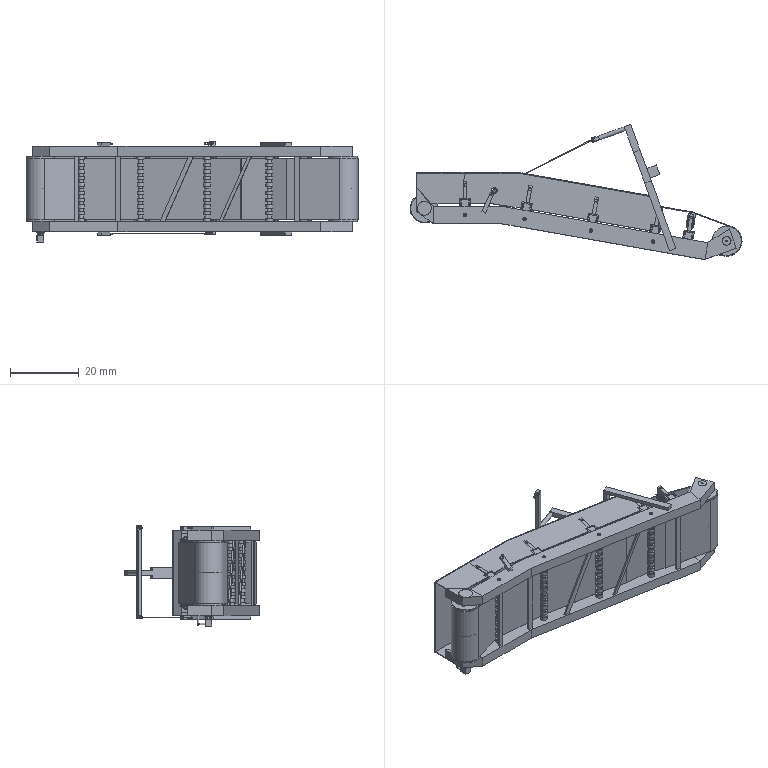Assembly | NX | mm | 27 component files | 141 solids | 1975 faces | box 96.68 x 39.38 x 29.23 mm | volume 7757 mm3 | plane 937 | cylinder 487 | cone 445 | sphere 86 | spline 14 | torus 6 | commonest cylinder face diameters 0.08 x104 0.1 x58 1.2 x41 2 x40 2.065 x35 1.51 x35 0.086 x27 0.8 x26
Bill of materials:
unnamed part 1 | 1 |  | Stepped solid cylinder: a larger central cylindrical body with a smaller coaxial cylindrical stub at each end.
unnamed part 2 | 5 |  | Rectangular open frame made of bar stock, with a long double-rib channel-like spine on one side, a fork-shaped connector at the ends, and a segmented, ribbed cylindrical member that bends in a shallow V/zigzag between the frame ends.
unnamed part 3 | 1 |  | Open framework of rectangular bars: a straight bar with small holes near both ends, joined by a stepped round/rectangular rod-and-block linkage to a C-shaped (three-sided) bar frame.
unnamed part 4 | 4 |  | Linked assembly-like shape: a U-bent round rod (hairpin loop) passes through a rectangular frame made of two flat bar plates joined by two round cross rods; a small pin is visible at the loop.
unnamed part 5 | 1 |  | Stepped cylinder: a large central cylindrical body with a smaller coaxial cylindrical stub at each end and a small axial hole through the center.
unnamed part 6 | 8 |  | Plain cylindrical sleeve/bushing-like tube with a concentric through-bore and flat ends.
unnamed part 7 | 4 |  | Slender stepped shaft with a regular series of evenly spaced larger-diameter collars/discs along its length, and stepped reduced-diameter ends.
unnamed part 8 | 1 |  | Long welded-frame-like structure of two parallel side plates with an angled (kinked) profile, joined by thin cross rods/bars and a solid web; it has round pivot holes at both ends, small holes, and stepped slot/notch features along the plates.
unnamed part 9 | 1 |  | Rectangular block body with stepped, smaller rectangular tiers on top, capped by a thin square flange plate with four corner holes and a larger central hole; two round rods leave the side, bend 90 degrees, and run upward parallel to each other.
unnamed part 10 | 1 |  | Thin-walled closed loop band: an elongated, slightly curved, rounded-end ring/strap profile extruded to a constant height, open on both faces.
Mates:
1. touch align | assembly face | model7 1
2. touch align | assembly face | model3 2
3. touch align | model3 2 | assembly face
4. touch align | assembly face | model3 1
5. touch align | assembly face | model3 1
6. touch align | HH 1 face | h5 5 face
7. touch align | HH 1 face | h5 5 face
8. touch align | HH 1 face | h5 4 face
9. touch align | HH 1 edge | h5 4 face
10. touch align | HH 1 face | h5 3 face
11. touch align | HH 1 face | h5 3 face
12. touch align | HH 1 face | h5 2 face
13. touch align | h5 2 face | HH 1 face
14. touch align | model5 1 face | h2 1 face
15. touch align | h5 1 face | HH 1 face
16. touch align | h5 1 face | HH 1 face
17. touch align | h5 1 face | HH 1 face
18. touch align | model2 4 face | HH 1 face
19. touch align | model2 4 face | HH 1 face
20. touch align | model2 3 face | HH 1 face
21. touch align | model2 3 face | HH 1 face
22. touch align | model2 2 face | HH 1 face
23. touch align | model2 2 face | HH 1 face
24. touch align | model2 1 face | HH 1 face
25. touch align | model2 1 face | HH 1 face
26. touch align | model11 4 face | HH 1 face
27. touch align | model11 4 face | HH 1 face
28. touch align | model11 3 face | HH 1 face
29. touch align | model11 3 face | HH 1 face
30. touch align | model11 2 face | HH 1 face
31. touch align | model11 2 face | HH 1 face
32. touch align | model11 1 face | HH 1 edge
33. touch align | model11 1 face | HH 1 face
34. concentric | model6 1 edge | HH 1